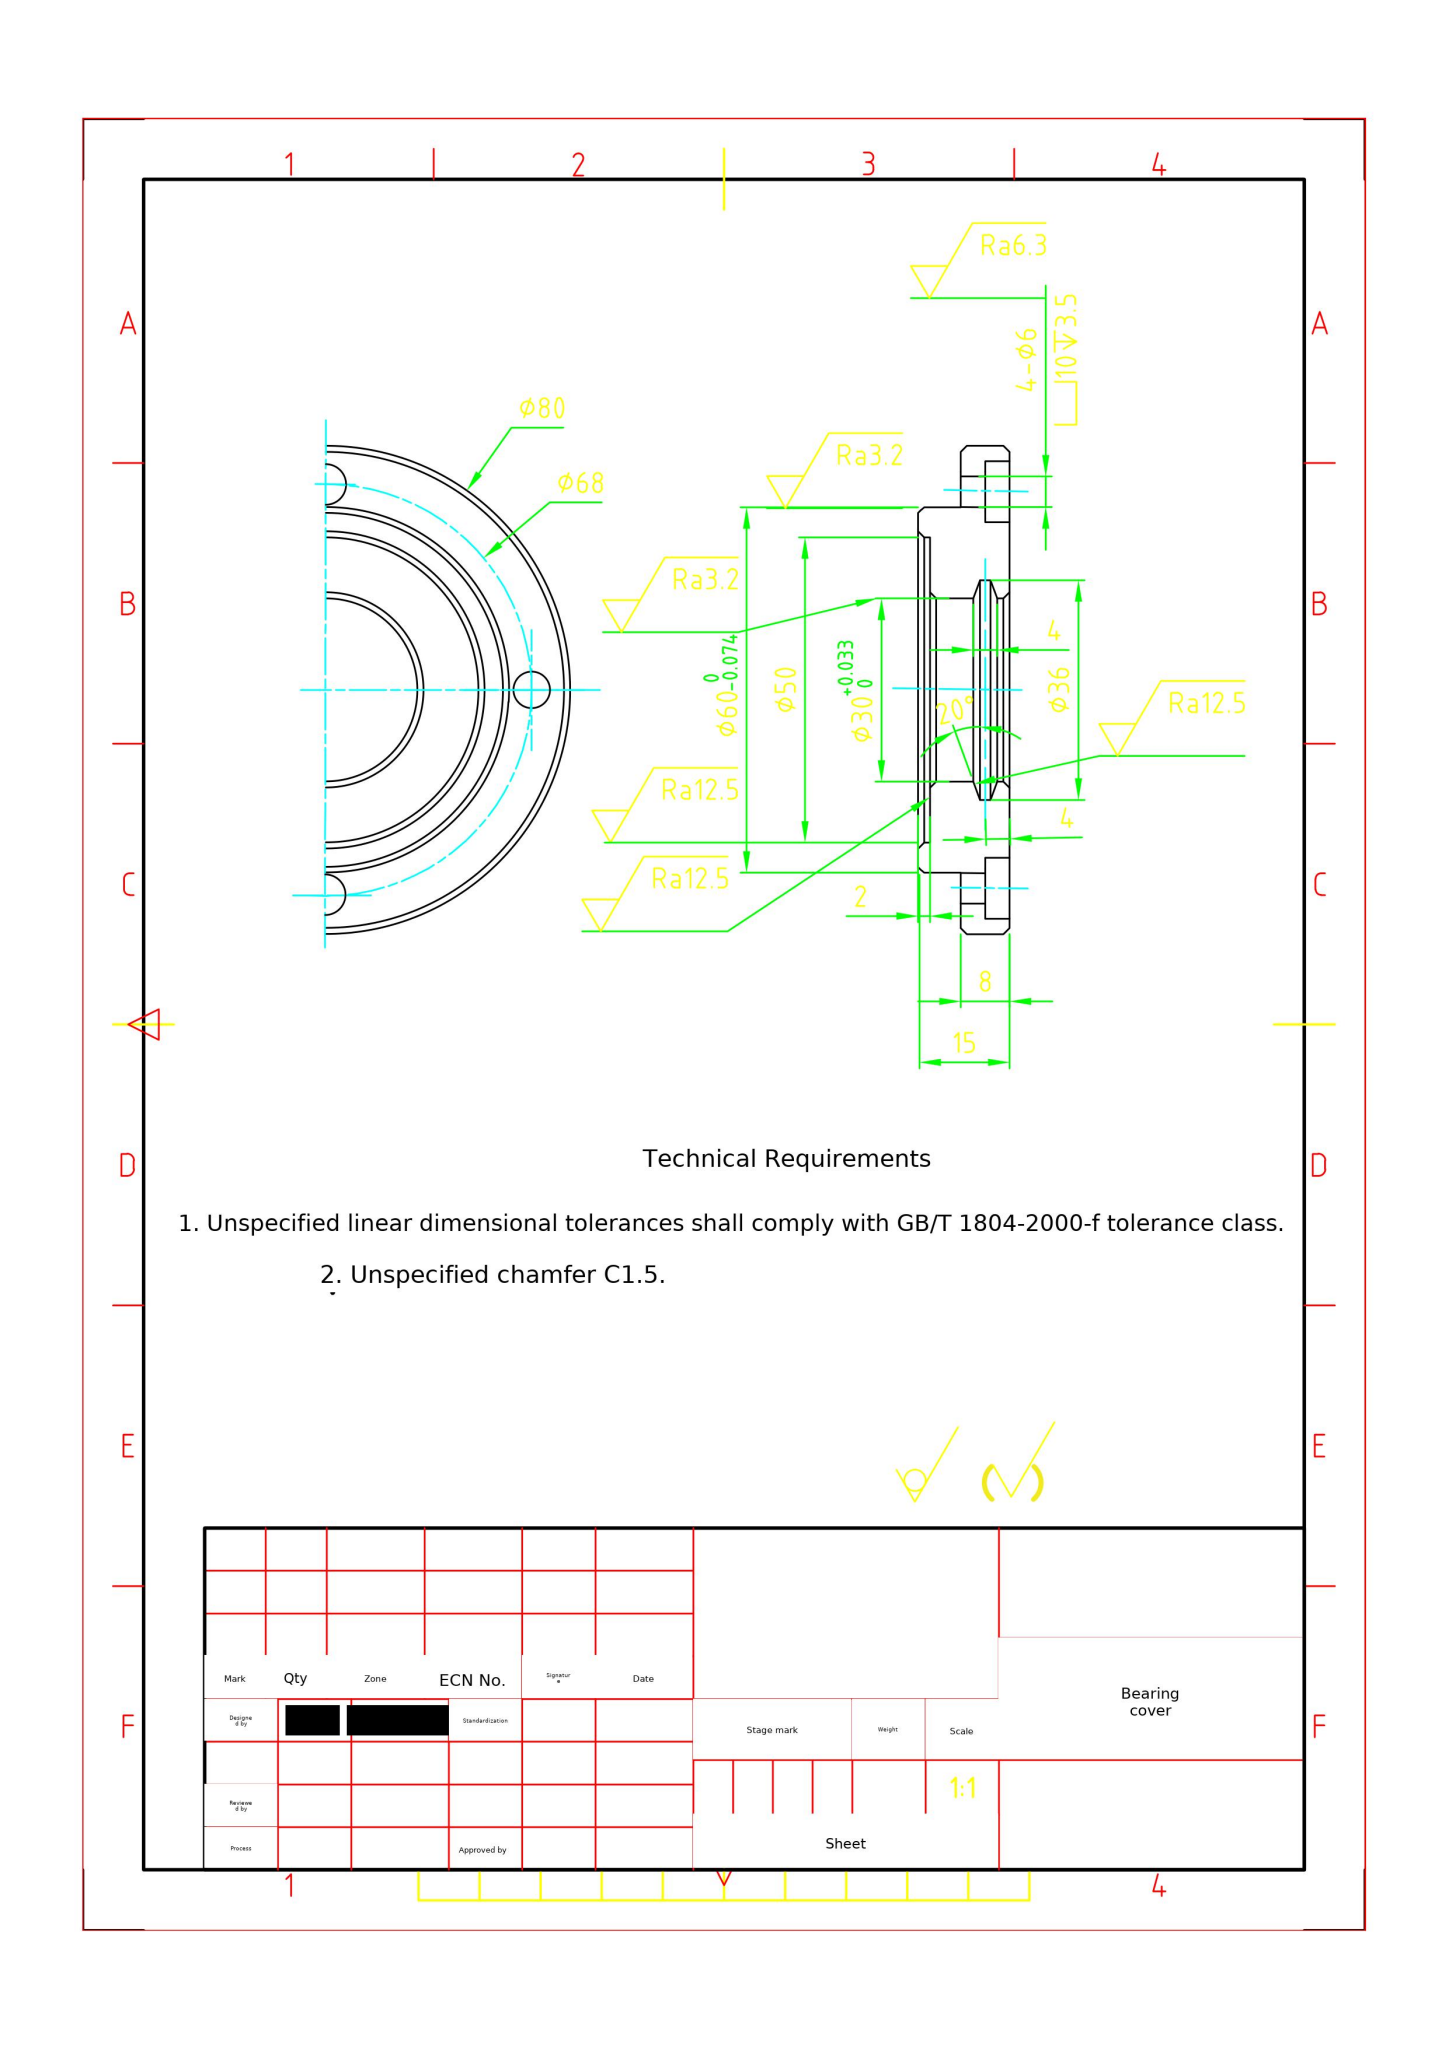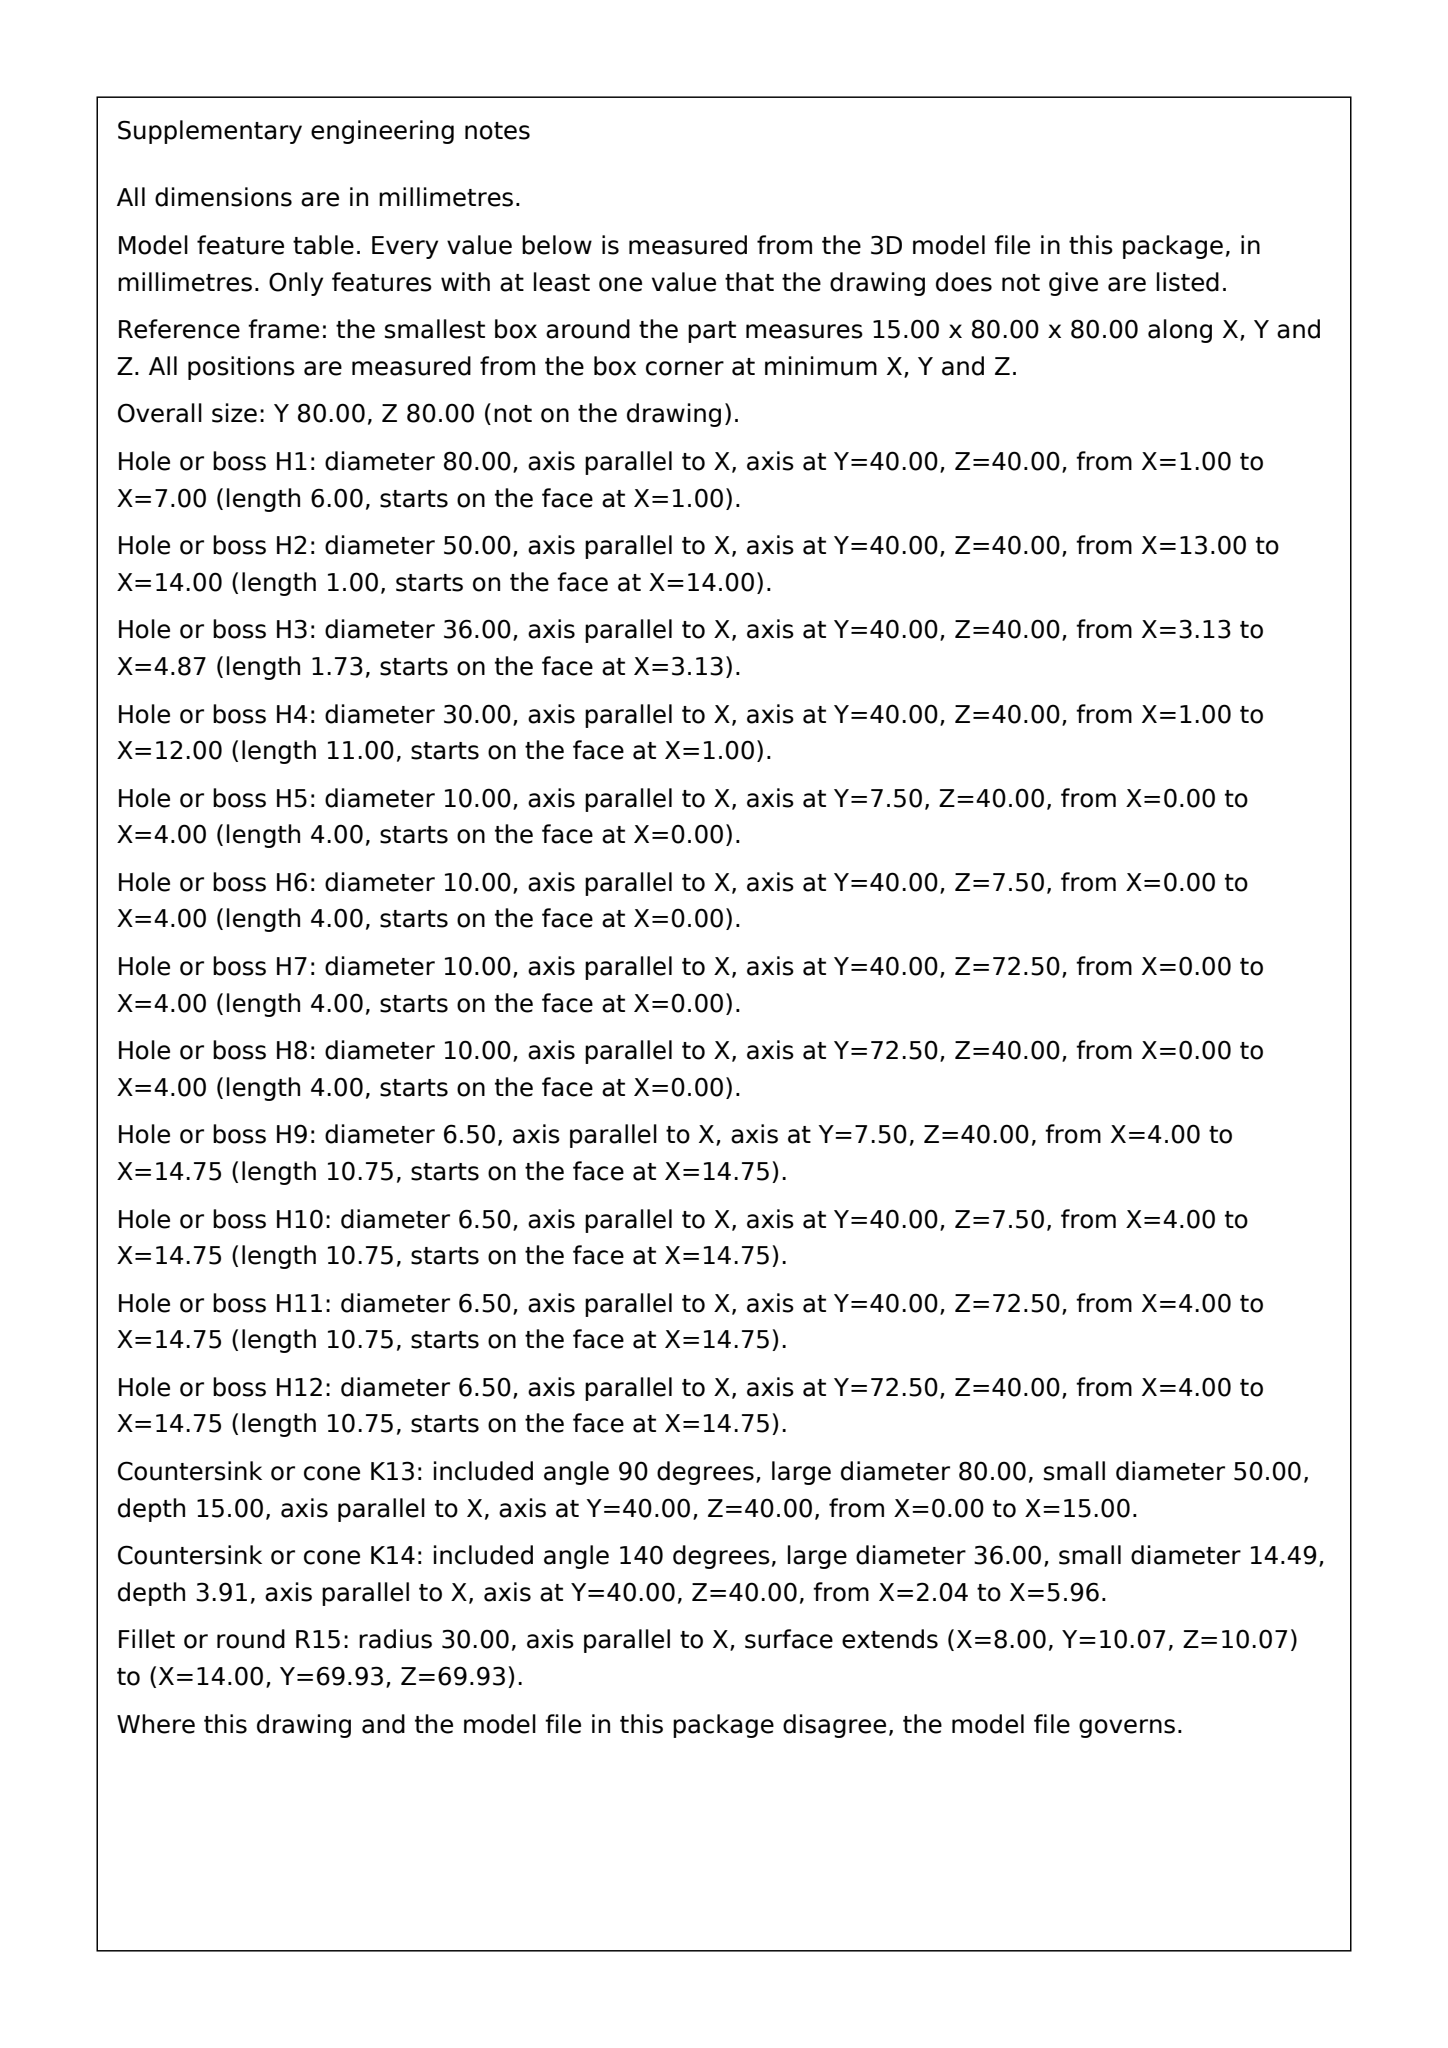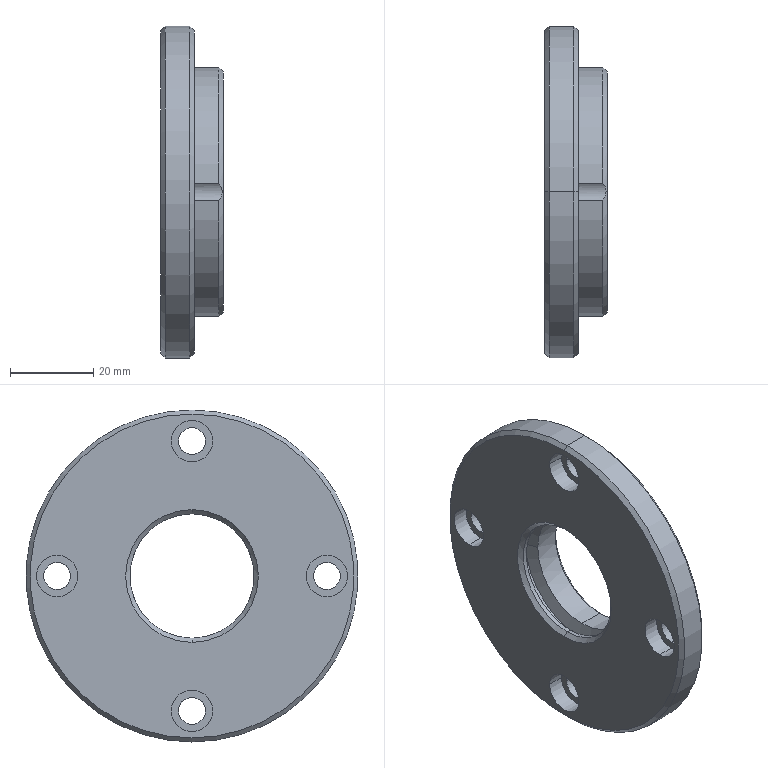Part | SolidWorks | mm | 1 solid | 54 faces | box 15 x 80 x 80 mm | volume 43663 mm3 | cylinder 30 | cone 16 | plane 8 | commonest cylinder face diameters 6.5 x8 10 x8 30 x4 60 x4 36 x2 50 x2 80 x2
build123d program:
from build123d import *

# Parameters (mm, degrees)
SKETCH2_R           = 40
SKETCH2_R_2         = 15
BOSS_EXTRUDE1_DEPTH = 15
SKETCH3_W           = 7
SKETCH3_H           = 10
SKETCH4_R           = 25
SKETCH4_R_2         = 10.804
CUT_EXTRUDE1_DEPTH  = 2
CHAMFER1_SIZE       = 1
CHAMFER2_SIZE       = 1
CHAMFER3_SIZE       = 1
SKETCH7_R           = 5
CUT_EXTRUDE2_DEPTH  = 4
CUT_EXTRUDE3_REACH  = 59.628
SKETCH9_R           = 3.25
CIRPATTERN1_COUNT   = 4


with BuildPart() as part:
    # Sketch2 → Boss-Extrude1 (new body)
    with BuildSketch(Plane(origin=(0, 0, 0), x_dir=(0, 0, -1), z_dir=(1, 0, 0))):
        Circle(SKETCH2_R)
        Circle(SKETCH2_R_2, mode=Mode.SUBTRACT)
    extrude(amount=BOSS_EXTRUDE1_DEPTH)

    # Sketch3 → Cut-Revolve1 (revolve, cut)
    with BuildSketch(Plane.XY, mode=Mode.PRIVATE) as cut_revolve1_sk:
        with Locations((11.5, 35)):
            Rectangle(SKETCH3_W, SKETCH3_H)
    revolve(cut_revolve1_sk.sketch.rotate(Axis((0, 0, 0), (1, 0, 0)), 90), axis=Axis((0, 0, 0), (1, 0, 0)), mode=Mode.SUBTRACT)

    # Sketch4 → Cut-Extrude1 (cut)
    with BuildSketch(Plane(origin=(15, 0, 0), x_dir=(0, 0, -1), z_dir=(1, 0, 0))):
        Circle(SKETCH4_R)
        Circle(SKETCH4_R_2, mode=Mode.SUBTRACT)
    extrude(amount=-CUT_EXTRUDE1_DEPTH, mode=Mode.SUBTRACT)

    # Chamfer1
    chamfer1_edges = [part.edges().sort_by_distance(p)[0] for p in [
        (8, 0, 40),
    ]]
    chamfer(chamfer1_edges, length=CHAMFER1_SIZE)

    # Chamfer2
    chamfer2_edges = [part.edges().sort_by_distance(p)[0] for p in [
        (15, 0, -30),
        (13, 0, 15),
        (15, 0, 25),
        (0, 0, 15),
    ]]
    chamfer(chamfer2_edges, length=CHAMFER2_SIZE)

    # Chamfer3
    chamfer3_edges = [part.edges().sort_by_distance(p)[0] for p in [
        (0, 0, 40),
    ]]
    chamfer(chamfer3_edges, length=CHAMFER3_SIZE)

    # Sketch5 → Cut-Revolve2 (revolve, cut)
    with BuildSketch(Plane.XY):
        Polygon((2, 14.883), (6, 14.883), (4.865, 18), (3.135, 18), align=None)
    revolve(axis=Axis((125, 0, 0), (-1, 0, 0)), mode=Mode.SUBTRACT)

    # Sketch7 → Cut-Extrude2 (cut)
    with BuildSketch(Plane.ZY):
        with Locations((0, 32.5)):
            Circle(SKETCH7_R)
    cut_extrude2 = extrude(amount=-CUT_EXTRUDE2_DEPTH, mode=Mode.SUBTRACT)

    # Sketch9 → Cut-Extrude3 (cut, up to next)
    with BuildSketch(Plane.ZY.offset(-4), mode=Mode.PRIVATE) as cut_extrude3_sk1:
        with Locations((0, 32.5)):
            Circle(SKETCH9_R)
    cut_extrude3_tool1 = extrude(cut_extrude3_sk1.sketch, amount=-CUT_EXTRUDE3_REACH, mode=Mode.PRIVATE) & part.part
    cut_extrude3 = cut_extrude3_tool1.solids().sort_by_distance((4, 32.5, 0))[0]
    add(cut_extrude3, mode=Mode.SUBTRACT)

    # CirPattern1: Cut-Extrude2, Cut-Extrude3 ×4 about axis
    cirpattern1_axis = Axis((0, 0, 0), (1, 0, 0))
    add([cut_extrude2.rotate(cirpattern1_axis, i * 360 / CIRPATTERN1_COUNT) for i in range(1, CIRPATTERN1_COUNT)], mode=Mode.SUBTRACT)
    add([cut_extrude3.rotate(cirpattern1_axis, i * 360 / CIRPATTERN1_COUNT) for i in range(1, CIRPATTERN1_COUNT)], mode=Mode.SUBTRACT)


solid = part.part